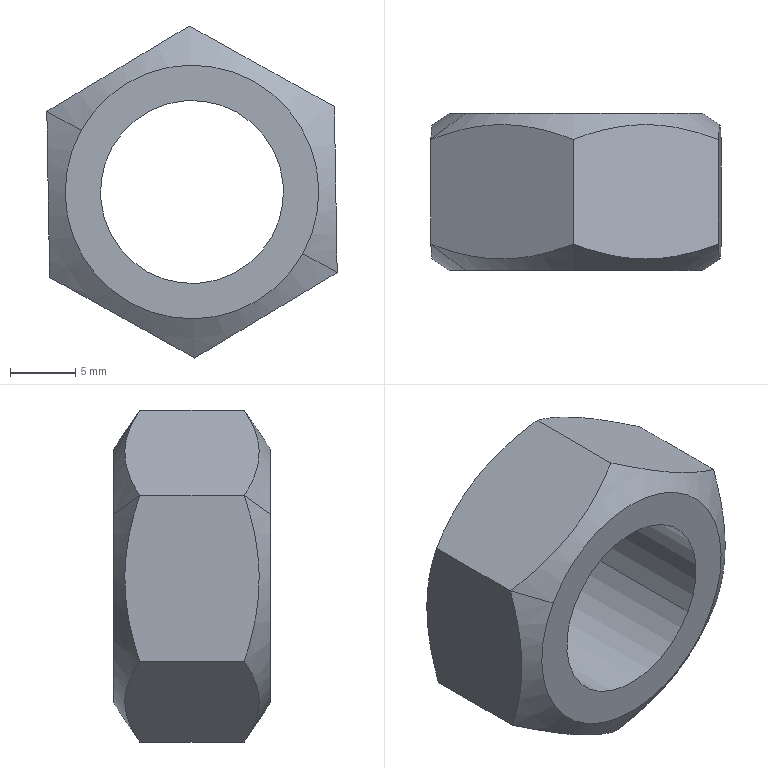Component | SolidWorks | M14Nut9.26-16 | 1 solid | 14 faces | volume 3014 mm3 | plane 8 | cone 4 | cylinder 2 | commonest cylinder face diameters 14 x2 | material AISI 1045 Steel, Cold Drawn